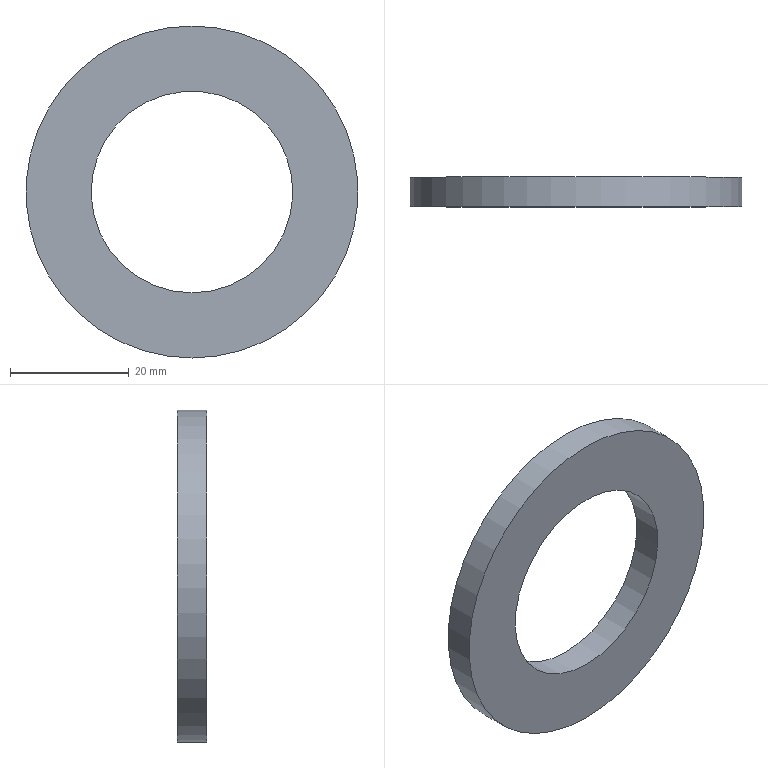Component | NX | GB-T848-2002_M33_2 | 1 solid | 4 faces | volume 7775 mm3 | cylinder 2 | plane 2 | commonest cylinder face diameters 56 x1 34 x1